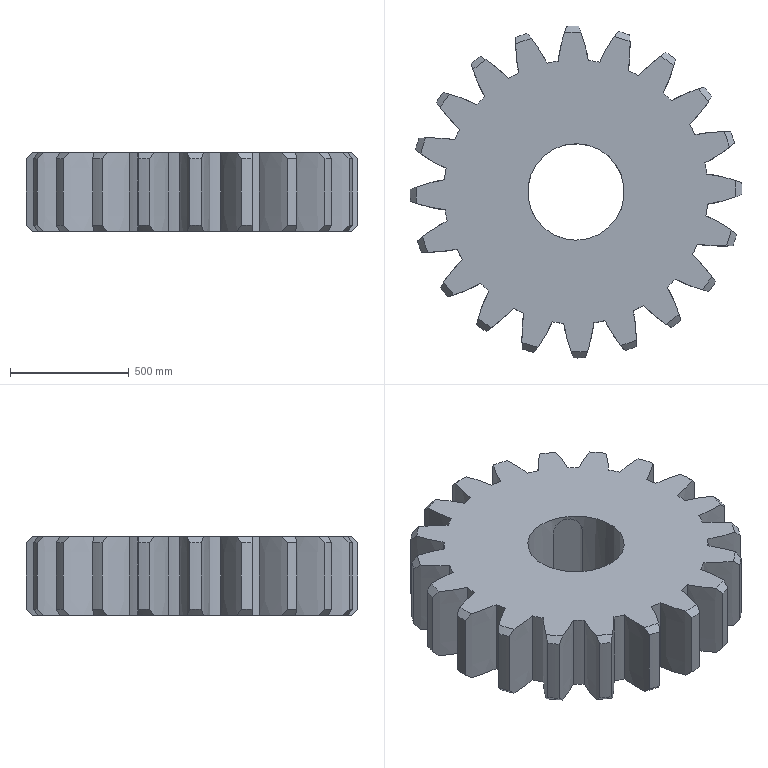Component | NX | 11 | 1 solid | 127 faces | volume 363860108 mm3 | cylinder 42 | other 40 | cone 40 | plane 5 | commonest cylinder face diameters 1111.25 x20 1397 x20 406.4 x1 127 x1